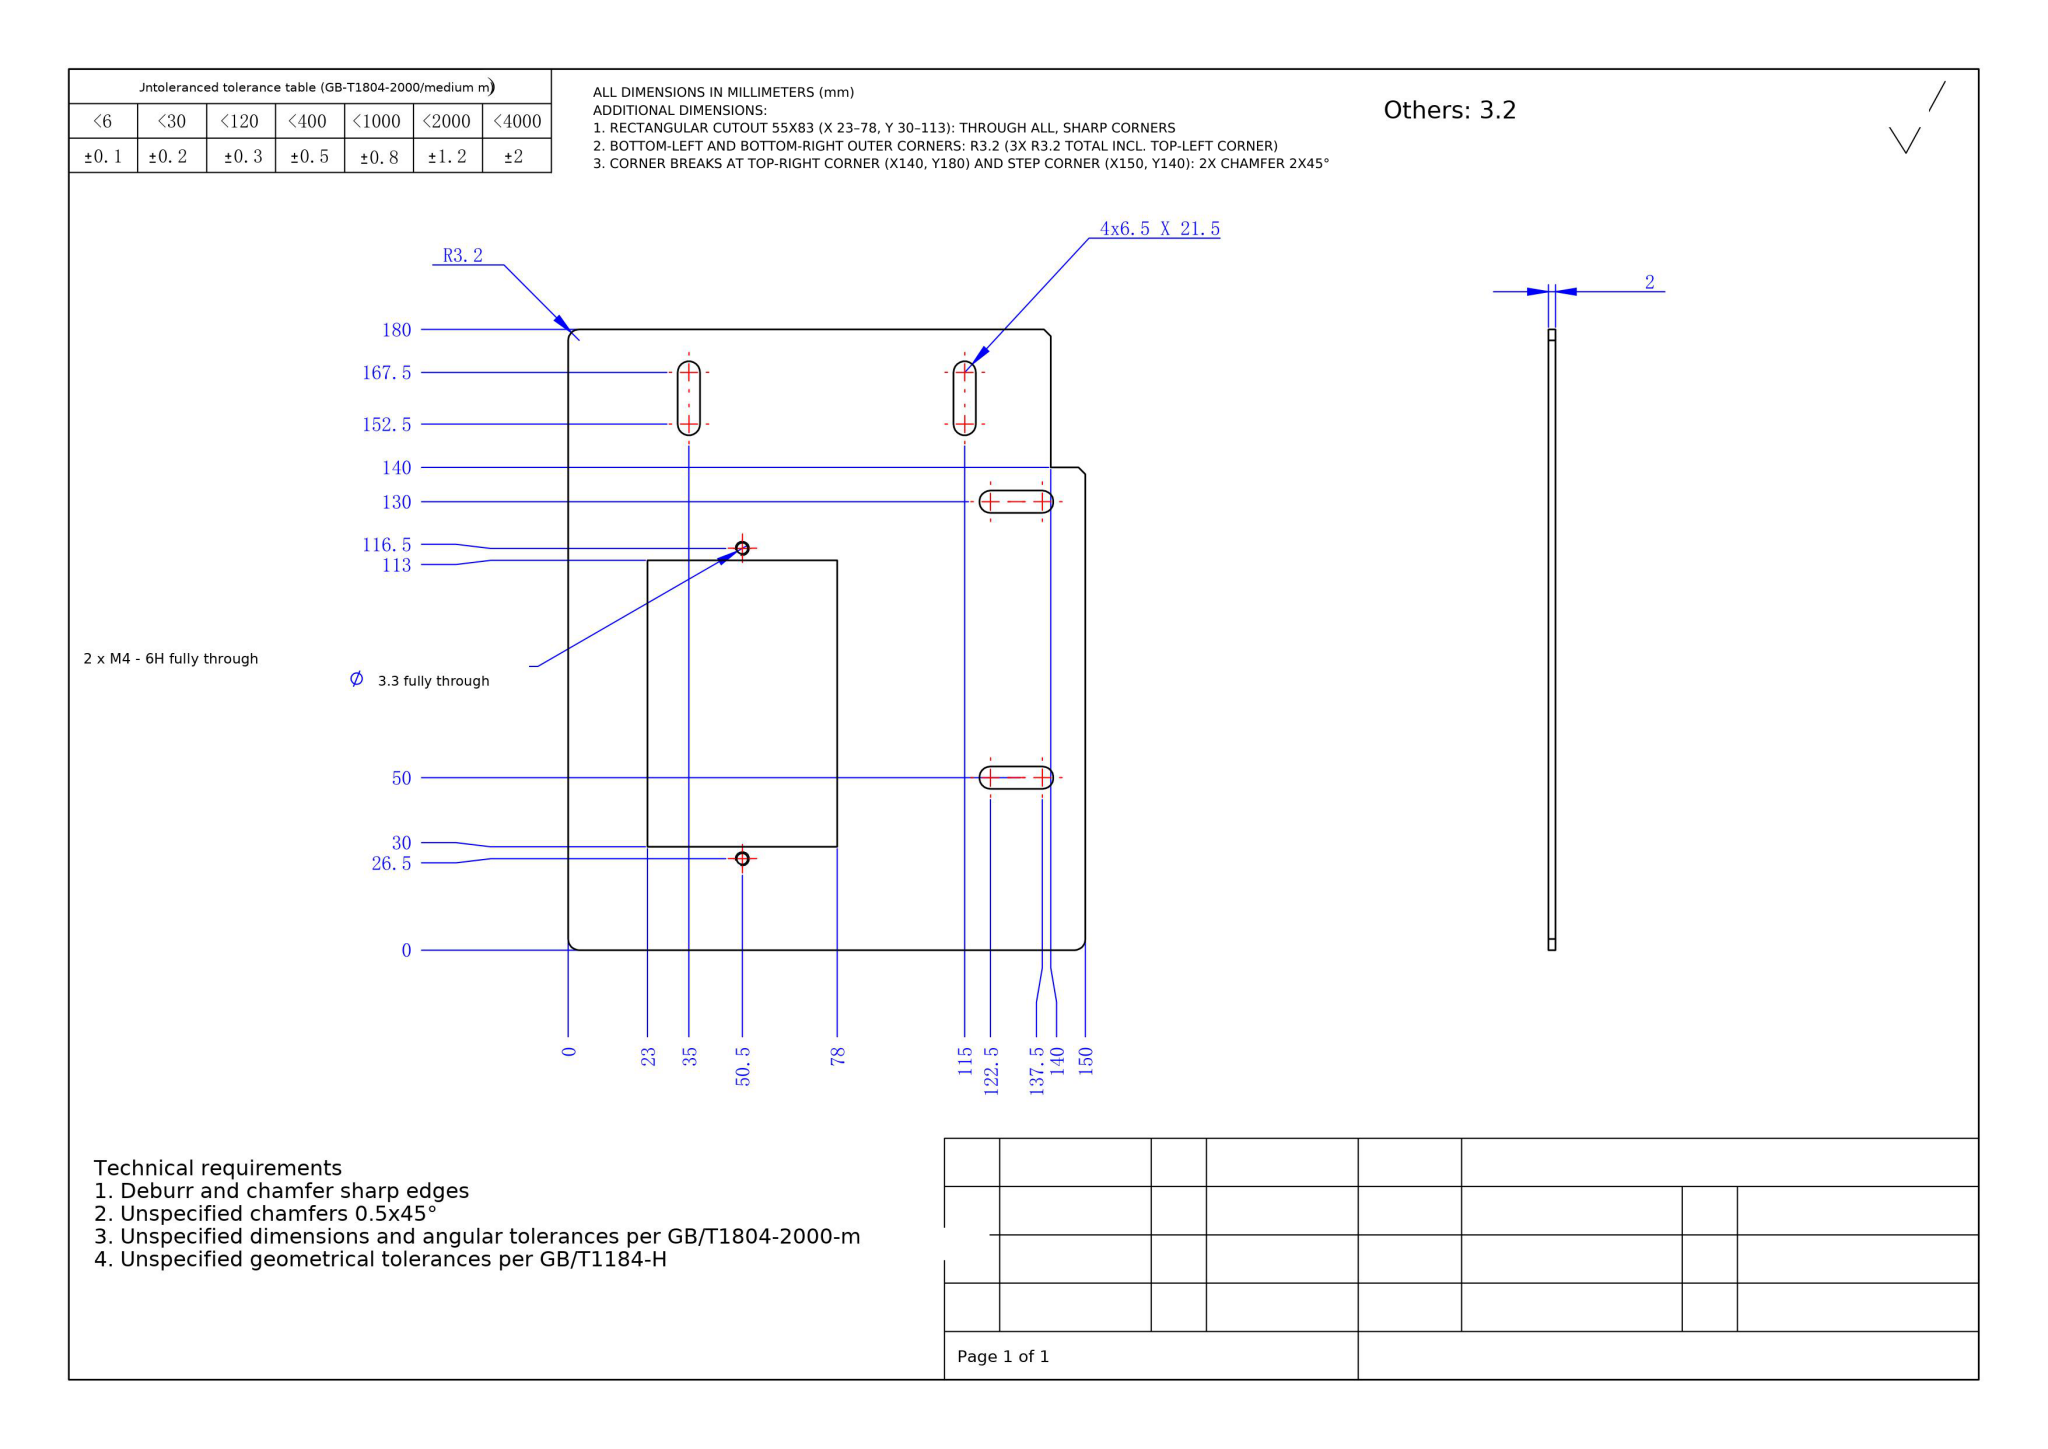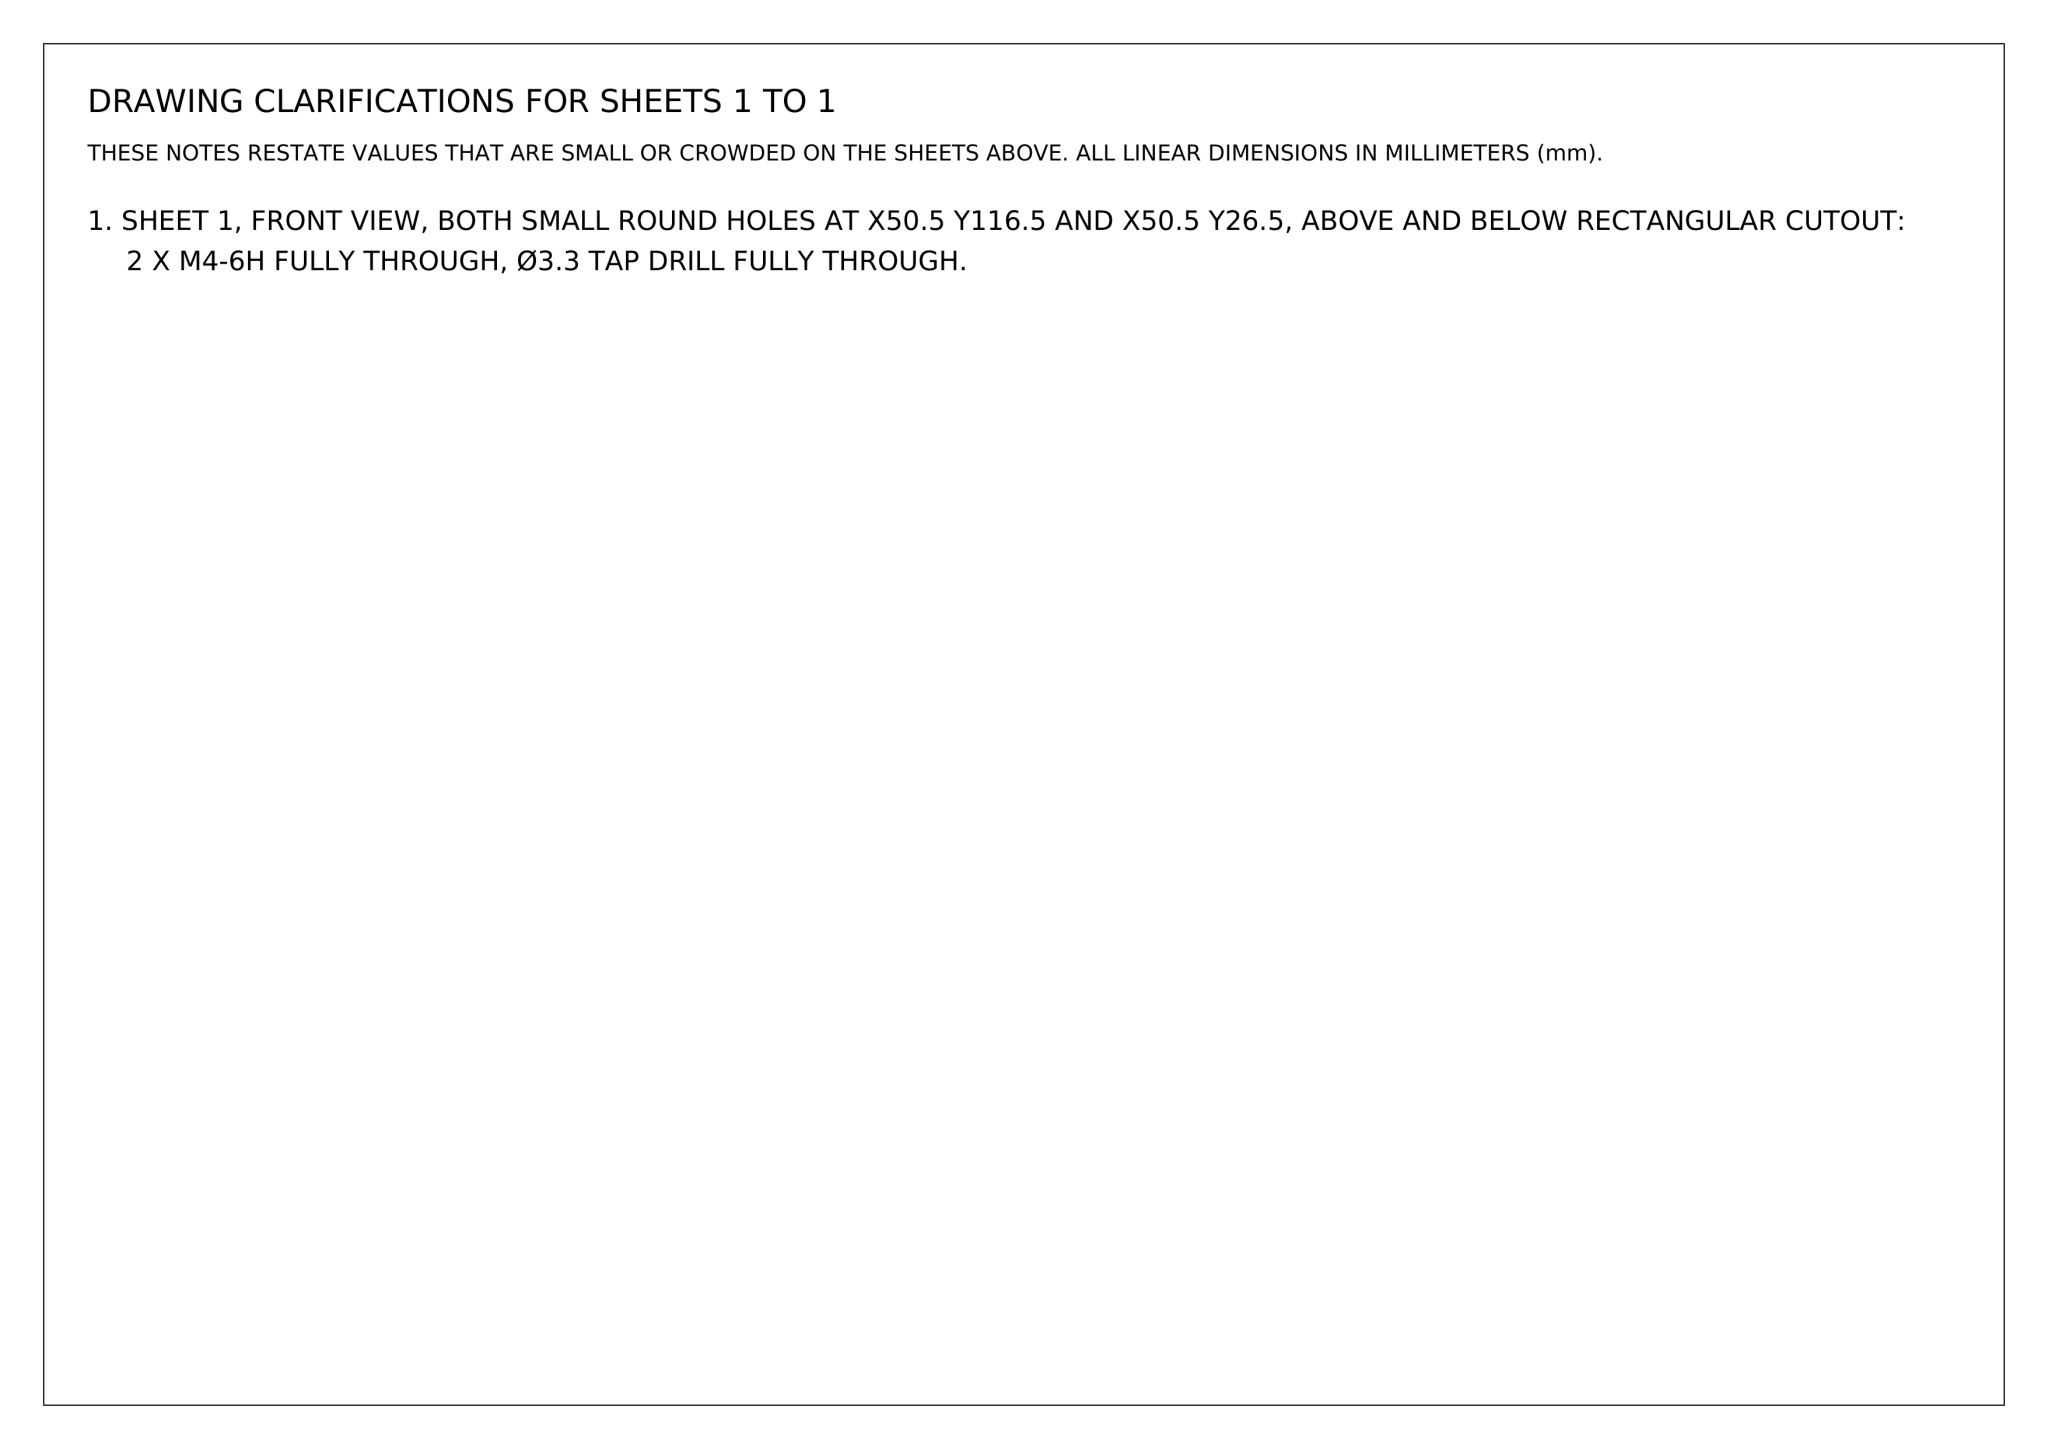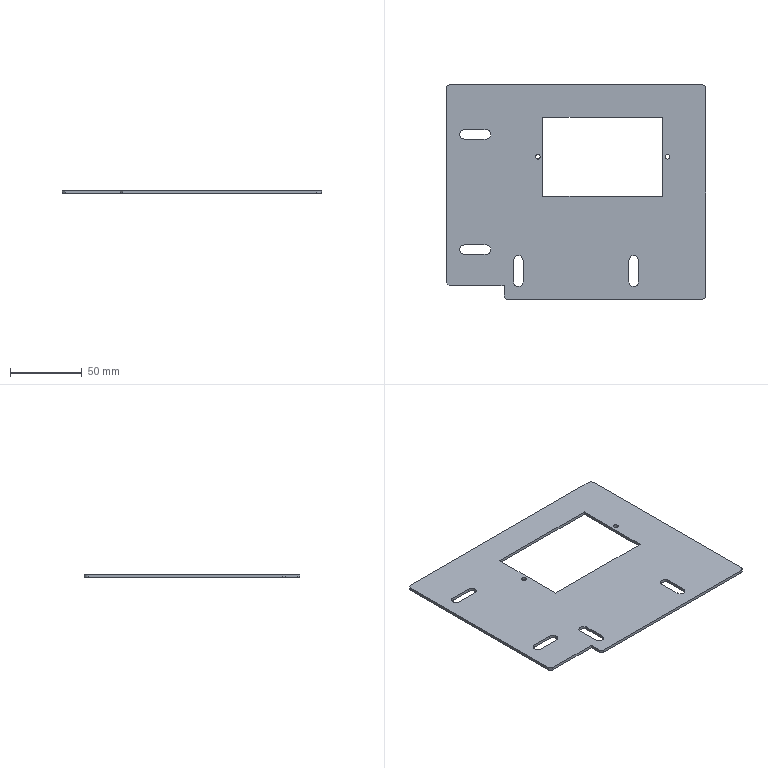Part | NX | mm | 1 solid | 39 faces | box 180 x 150 x 2 mm | volume 42969 mm3 | plane 22 | cylinder 17 | commonest cylinder face diameters 6.5 x10 3.3 x4 6.4 x3